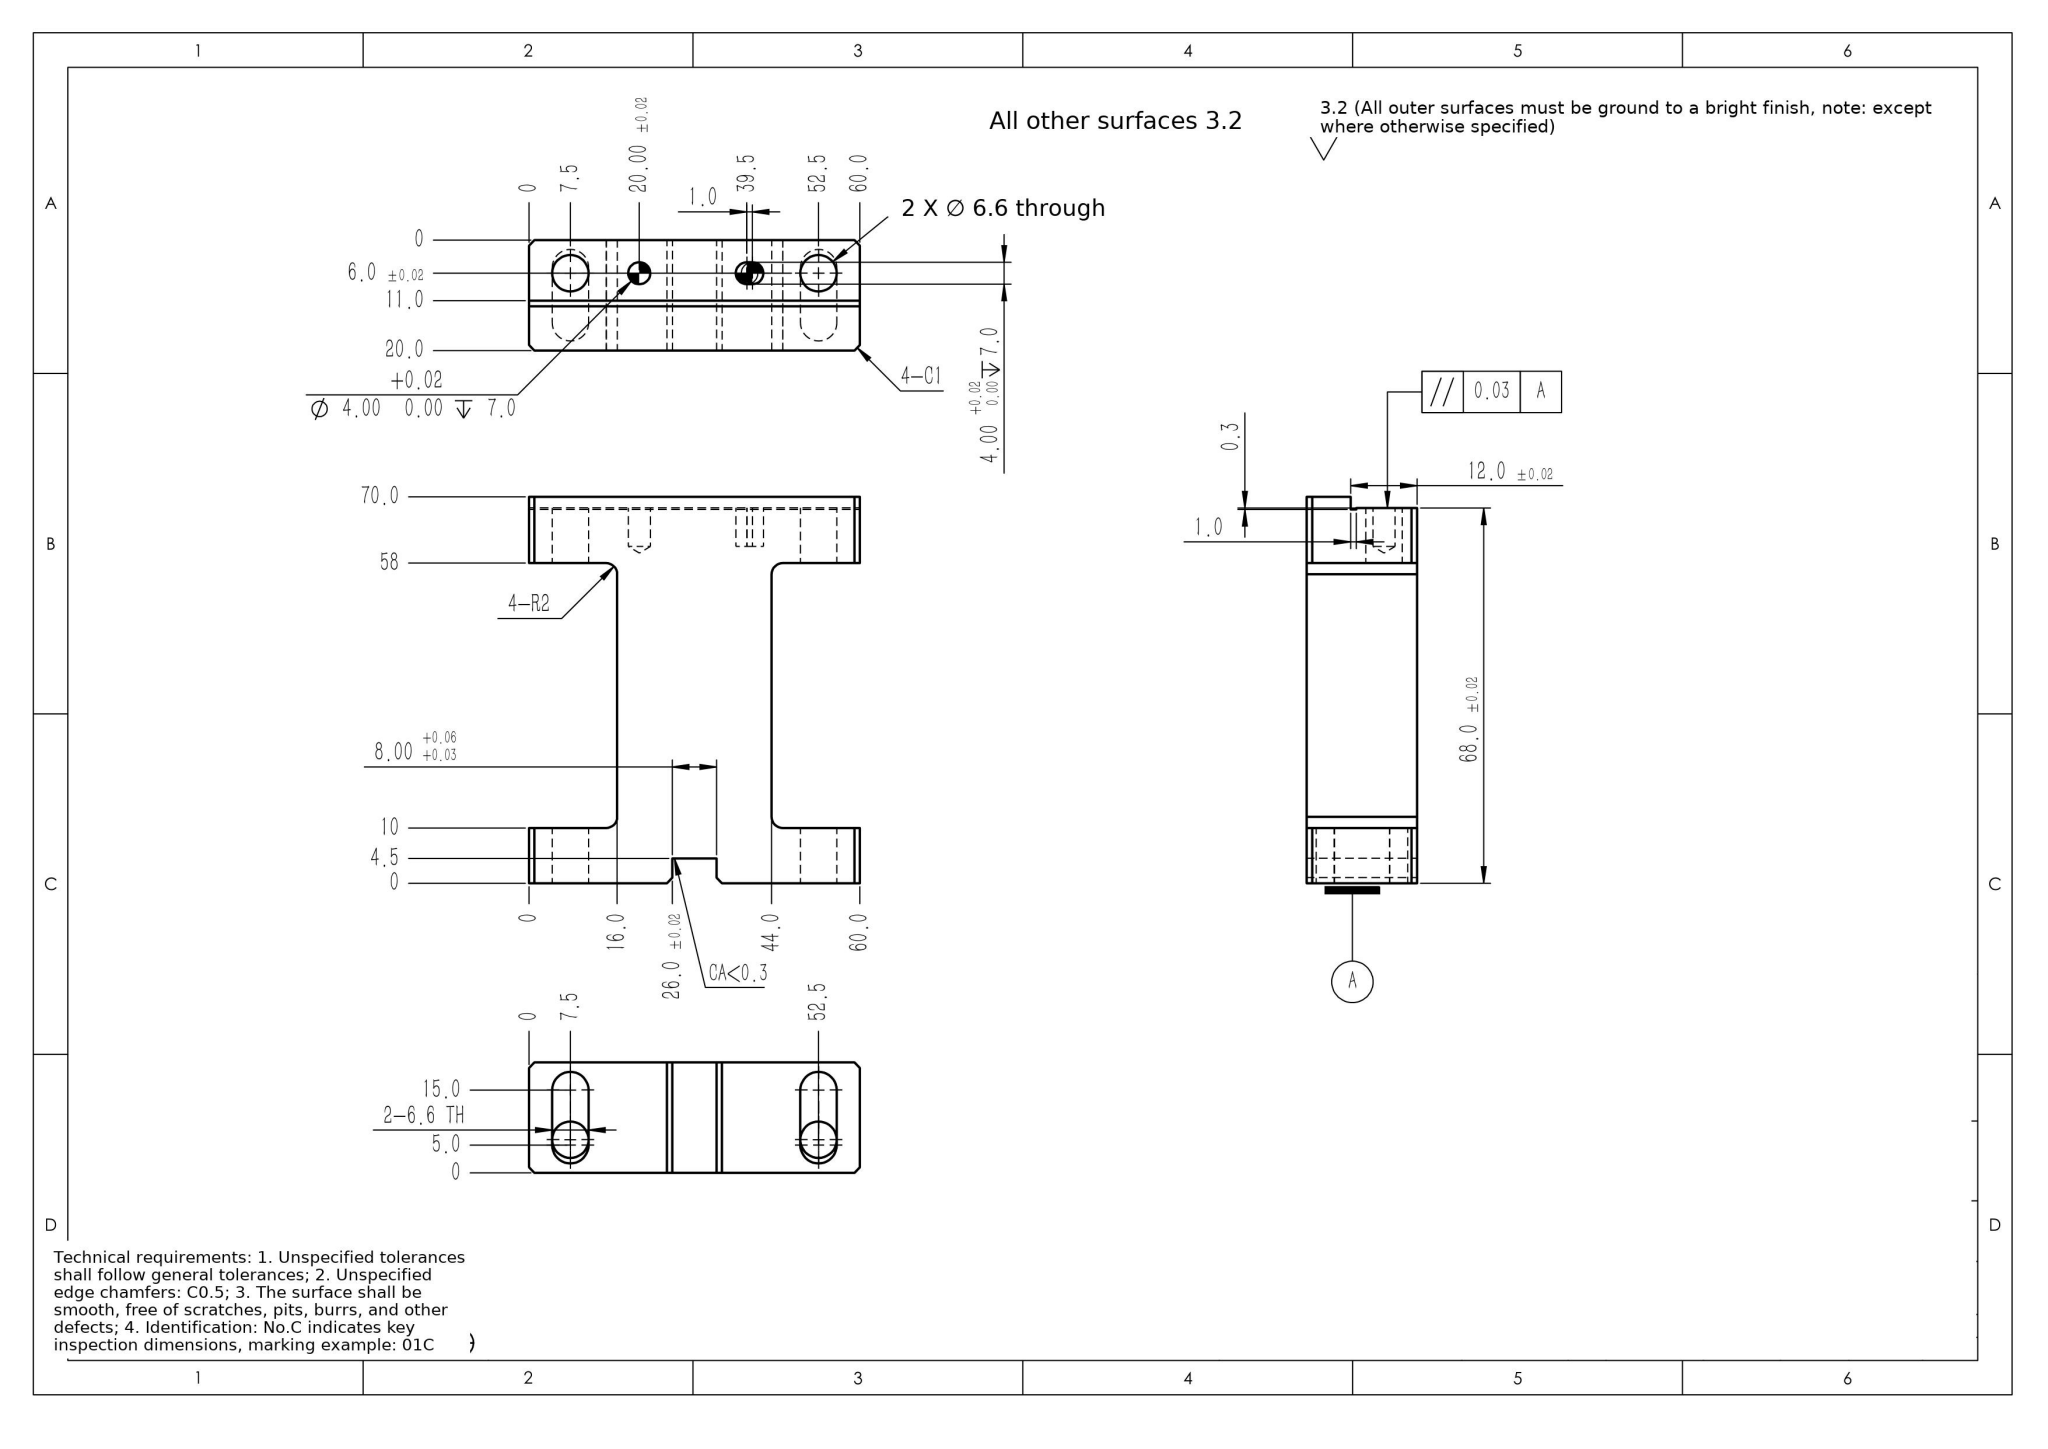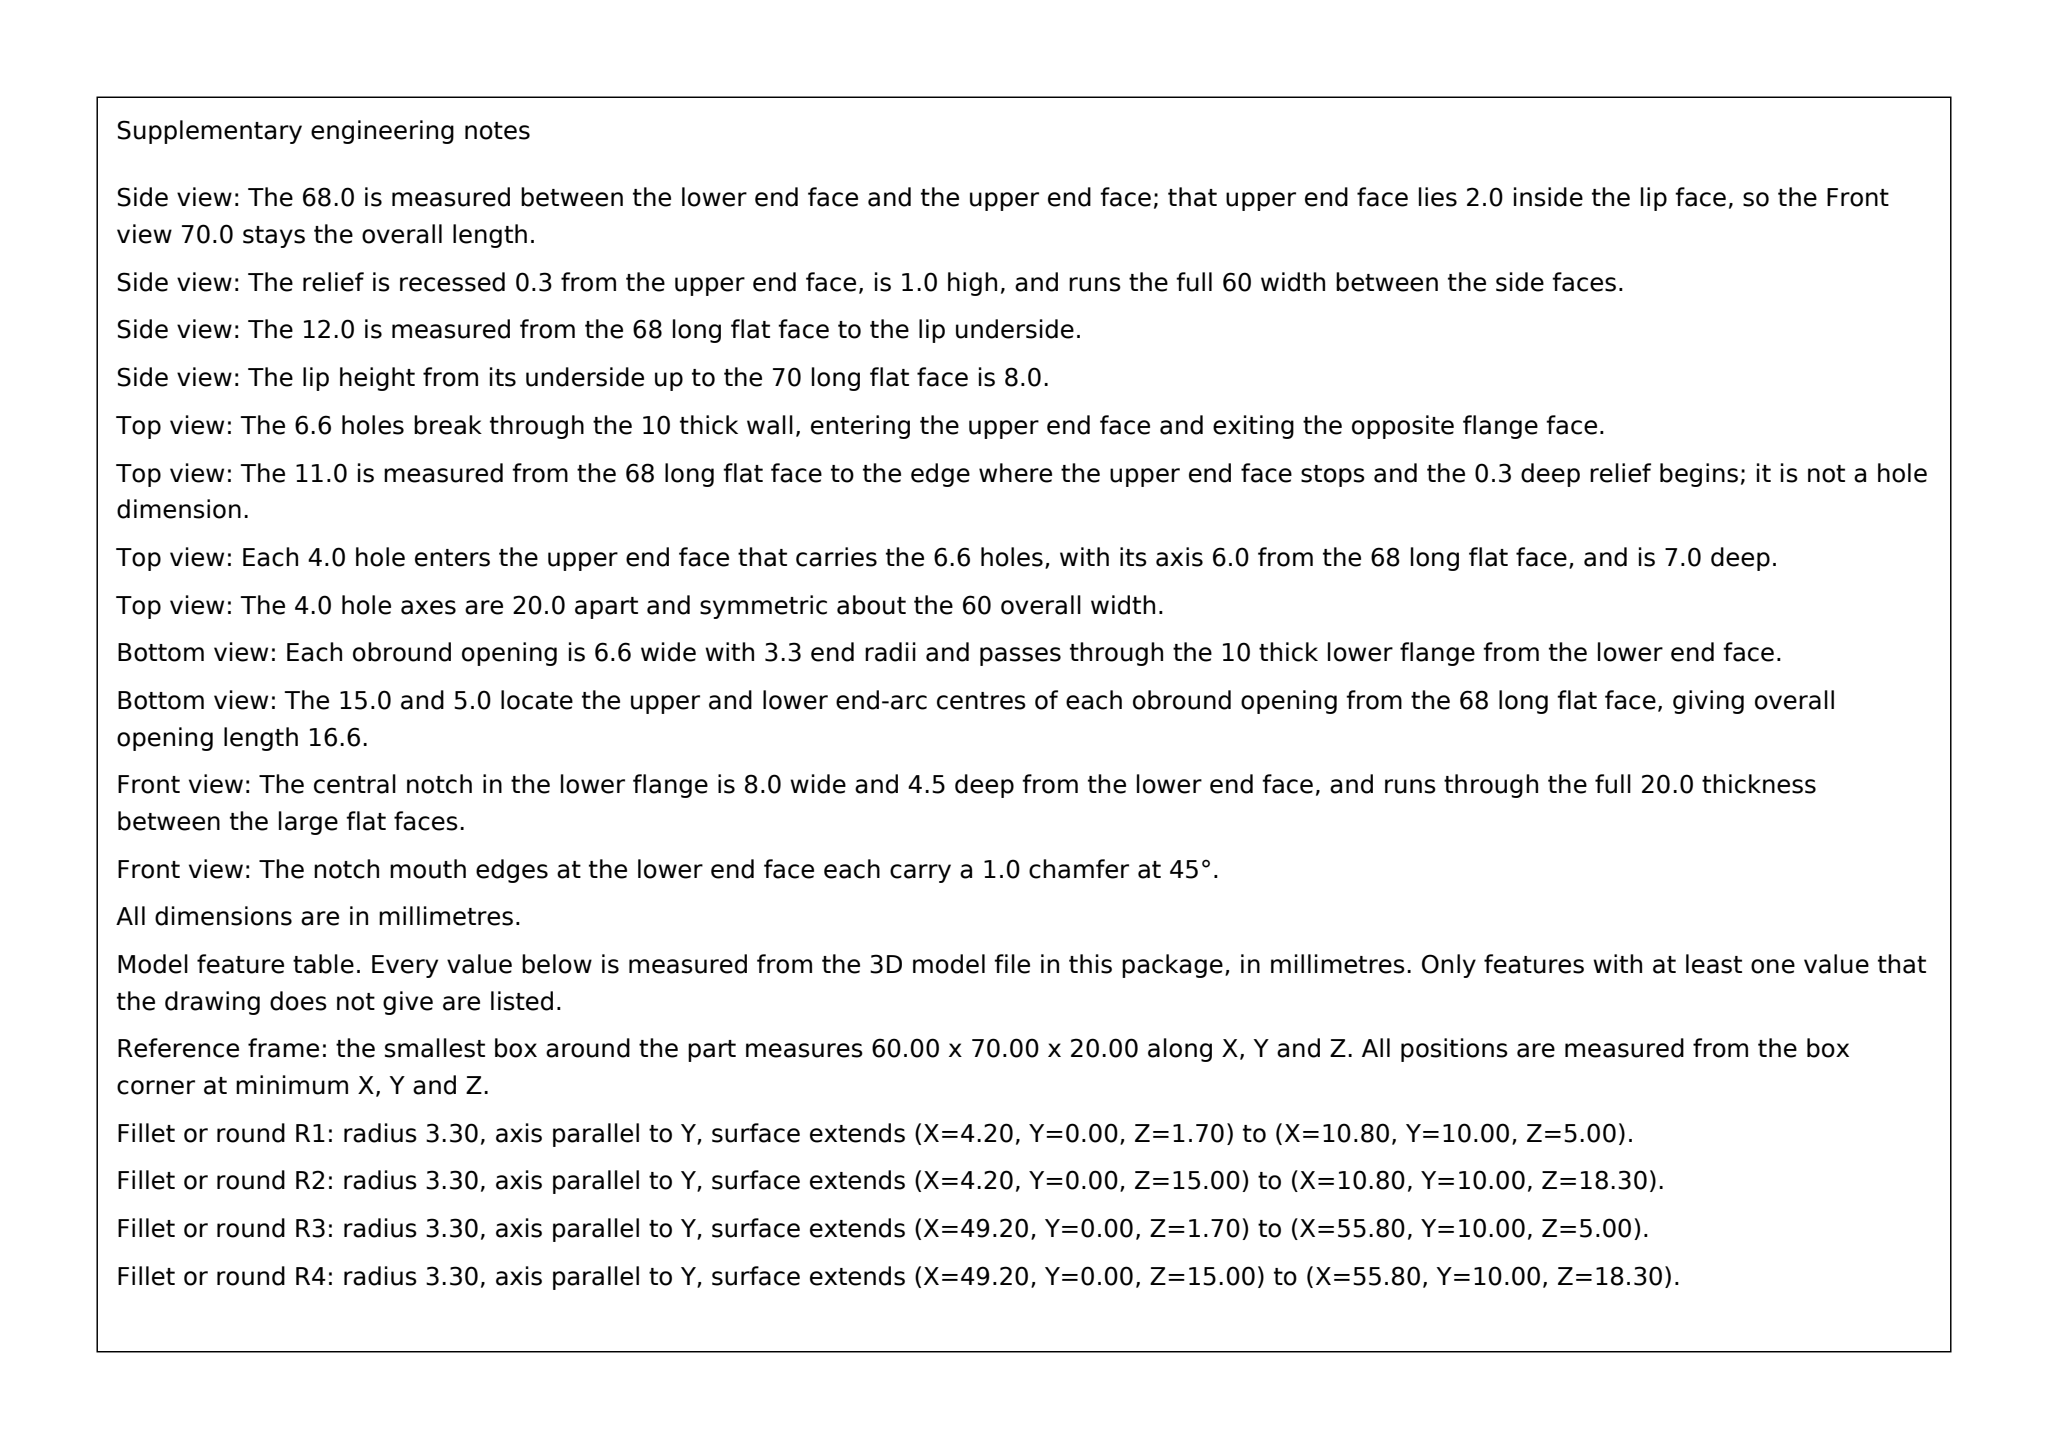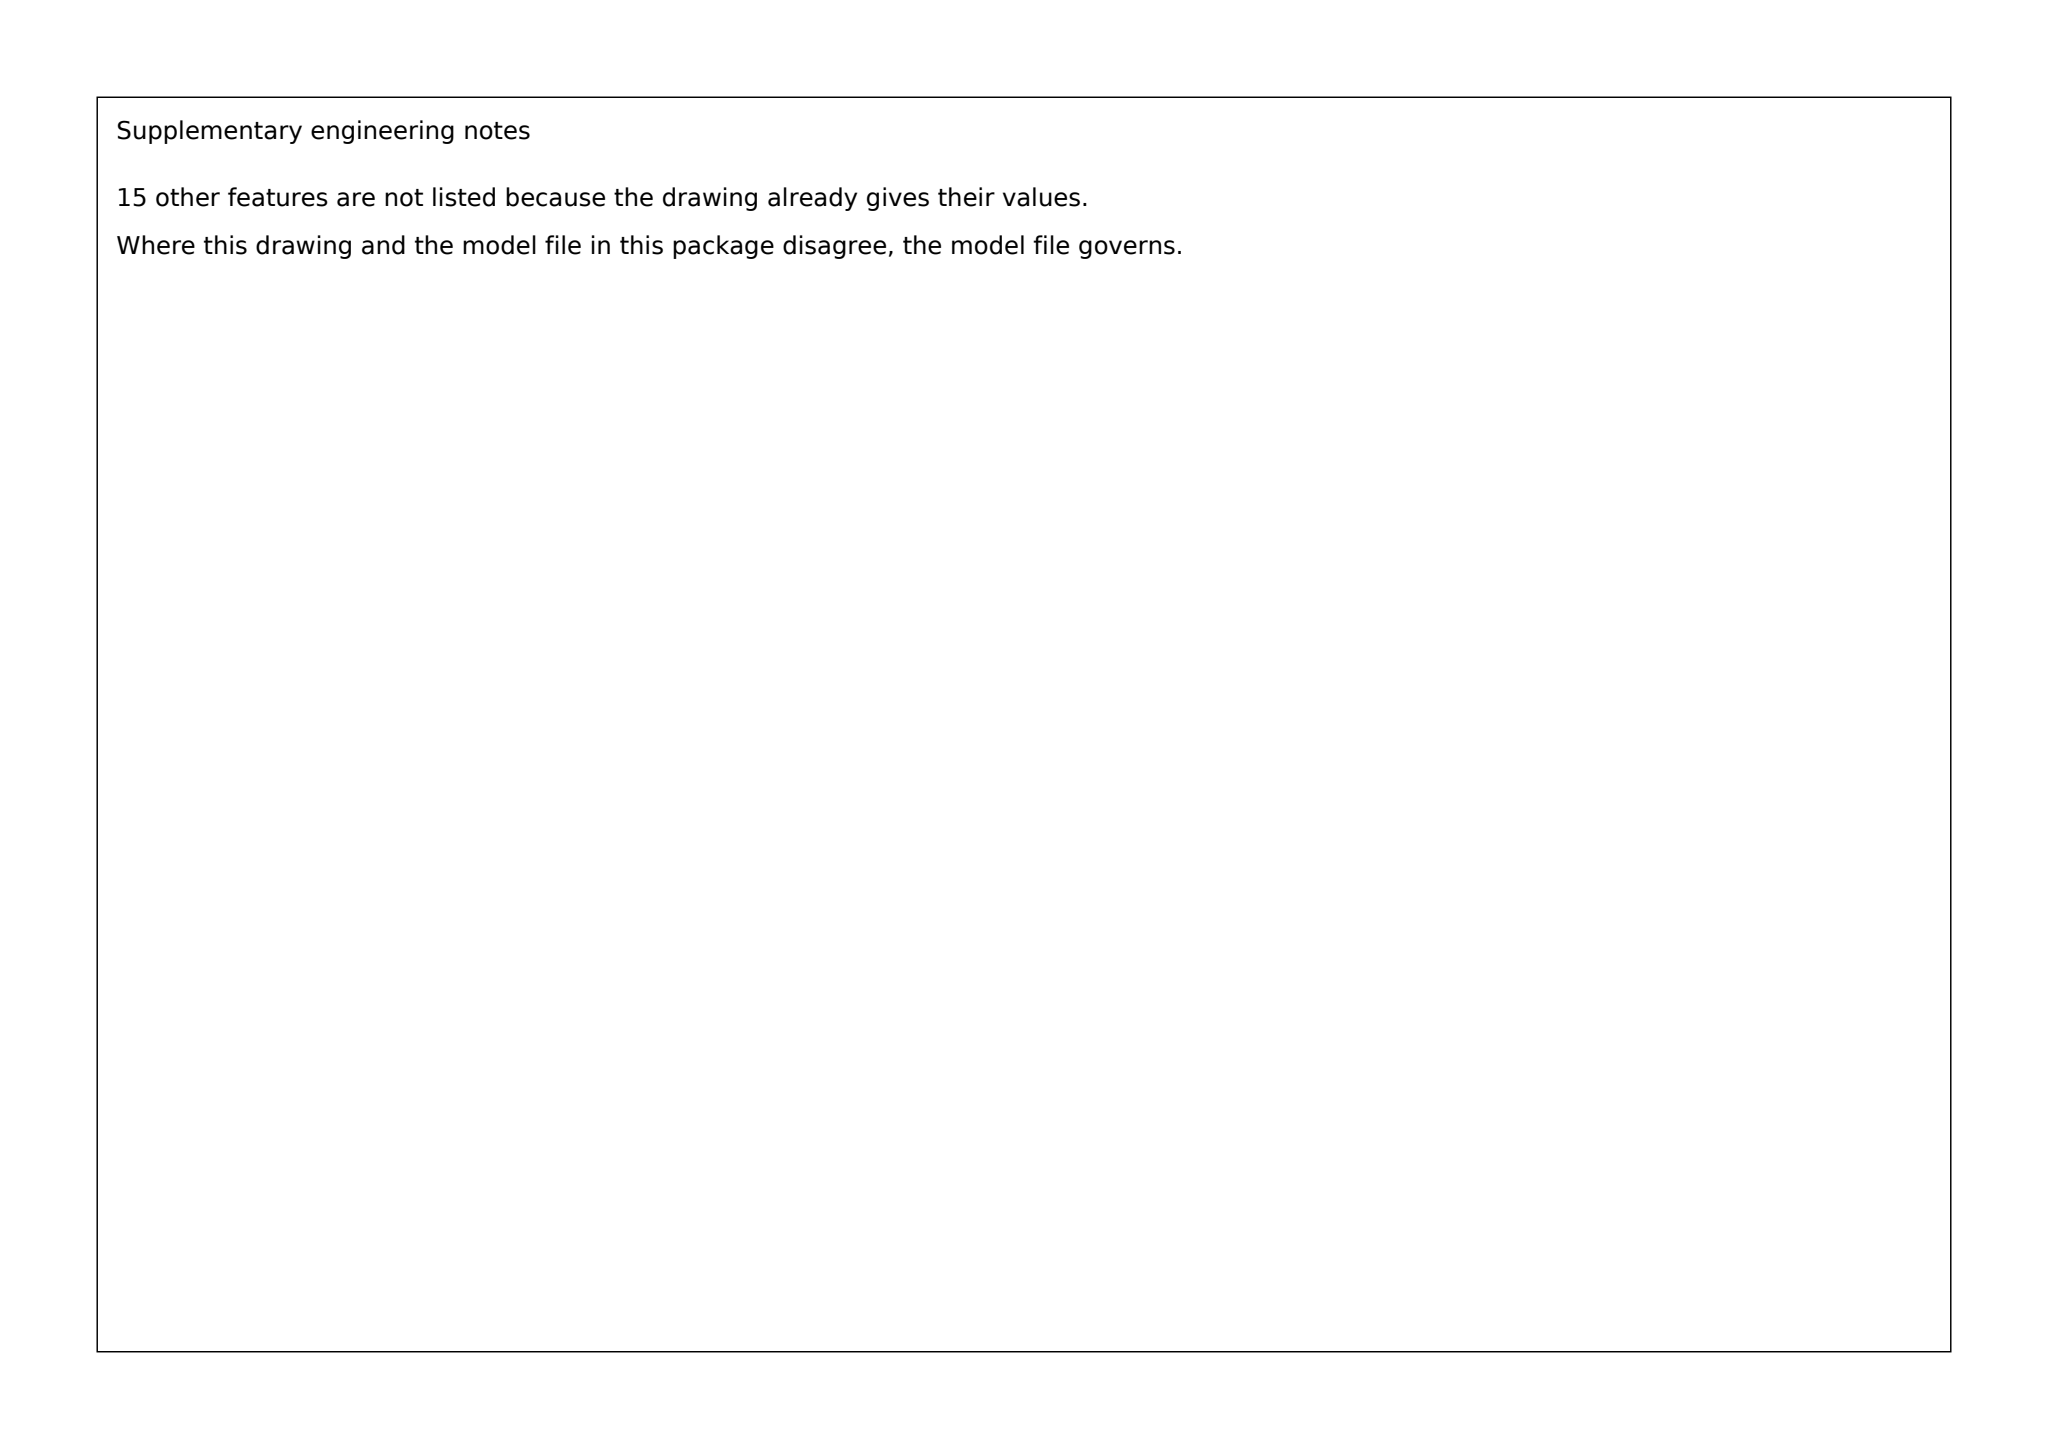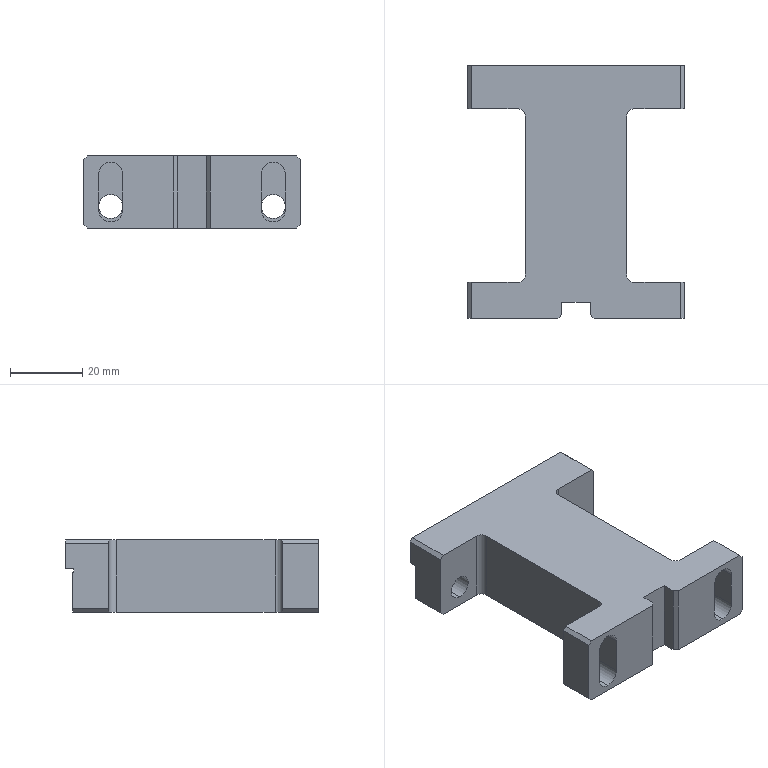Part | SolidWorks | mm | 1 solid | 59 faces | box 60 x 70 x 20 mm | volume 48211 mm3 | plane 39 | cylinder 18 | cone 2 | commonest cylinder face diameters 6.6 x10 4 x8
Drawing notes:
4X Ø4.0 THRU; X=14.0 & 46.0, Y=12.0 & 56.0 FROM 0 DATUM | from the solid: cylinders dia 4.0 axis z at (14,12),(14,56),(46,12),(46,56), length 20
4X Ø4.0 Z-AXIS HOLES THRU ALL (20.0 THK), NO C'BORE | from the solid: dia 4.0 axis z cylinders length 20.0 = full bbox z 20.0; no counterbore planes/cones on z axis
2X Ø4.00 +0.02/0 DP 7.0 AT X=20.00 & SLOT X=39.5/40.5, Z=6.0 | from the solid: dia 4.0 axis y at x=20.0 z=6.0 L7.0 (x2) and x=39.5/40.5 z=6.0 L7.0; cones 118° ref dia 4.0 x2
SLOT Ø4.00 +0.02/0 x 1.0 LG DP 7.0, CTRS X=39.5 & 40.5, Z=6.0 | from the solid: two dia 4.0 y-axis cylinders at x=39.5 and 40.5, z=6.0, length 7.0 (1.0 ctr spacing)
0.3 DEEP STEP ON TOP FACE FULL WIDTH, X=0 TO 60.0 | from the solid: y planes 68.0 and 67.7 (0.3 apart); no intermediate x planes besides slot walls, bbox x=60.0
build123d program:
from build123d import *

# Parameters (mm, degrees)
SKETCH2_W                      = 60
SKETCH2_H                      = 68
BOSS_EXTRUDE1_DEPTH            = 20
SKETCH3_W                      = 16
SKETCH3_H                      = 48
CUT_EXTRUDE1_DEPTH             = 20
F_6_6_6_6_DIAMETER_HOLE2_D     = 6.6
F_6_6_6_6_DIAMETER_HOLE2_DEPTH = 10
SIZE_MM_DOWEL_PIN_HOLE_1_D     = 4
SIZE_MM_DOWEL_PIN_HOLE_1_DEPTH = 7
SIZE_MM_DOWEL_PIN_HOLE_1_TIP   = 1.202
CUT_EXTRUDE2_DEPTH             = 7
SKETCH18_W                     = 8
SKETCH18_H                     = 4.5
CUT_EXTRUDE5_DEPTH             = 50.558
SKETCH19_W                     = 60
SKETCH19_H                     = 8
BOSS_EXTRUDE4_DEPTH            = 2
SKETCH20_W                     = 1
SKETCH20_H                     = 0.3
CUT_EXTRUDE6_DEPTH             = 73.774
CUT_EXTRUDE7_REACH             = 80.74
CHAMFER1_SIZE                  = 1
FILLET1_R                      = 2


with BuildPart() as part:
    # Sketch2 → Boss-Extrude1 (new body)
    with BuildSketch(Plane.XY):
        Rectangle(SKETCH2_W, SKETCH2_H)
    extrude(amount=BOSS_EXTRUDE1_DEPTH)

    # Sketch3 → Cut-Extrude1 (cut)
    with BuildSketch(Plane.XY.offset(20)):
        with Locations((-22, 0)):
            Rectangle(SKETCH3_W, SKETCH3_H)
        with Locations((22, 0)):
            Rectangle(SKETCH3_W, SKETCH3_H)
    extrude(amount=-CUT_EXTRUDE1_DEPTH, mode=Mode.SUBTRACT)

    # 6.6 _6.6_ Diameter Hole2
    with Locations(Plane(origin=(0, 34, 0), x_dir=(1, 0, 0), z_dir=(0, 1, 0))):
        with Locations((-22.5, -6), (22.5, -6)):
            Hole(F_6_6_6_6_DIAMETER_HOLE2_D / 2, depth=F_6_6_6_6_DIAMETER_HOLE2_DEPTH)

    # Size mm Dowel Pin Hole 1
    with Locations(Plane(origin=(0, 34, 0), x_dir=(1, 0, 0), z_dir=(0, 1, 0))):
        with Locations((-10, -6)):
            Hole(SIZE_MM_DOWEL_PIN_HOLE_1_D / 2, depth=SIZE_MM_DOWEL_PIN_HOLE_1_DEPTH)
            with Locations((0, 0, -(SIZE_MM_DOWEL_PIN_HOLE_1_DEPTH + SIZE_MM_DOWEL_PIN_HOLE_1_TIP / 2))):  # 118° drill point
                Cone(0, SIZE_MM_DOWEL_PIN_HOLE_1_D / 2, SIZE_MM_DOWEL_PIN_HOLE_1_TIP, mode=Mode.SUBTRACT)

    # Sketch8 → Cut-Extrude2 (cut)
    with BuildSketch(Plane(origin=(0, 34, 0), x_dir=(1, 0, 0), z_dir=(0, 1, 0))):
        with BuildLine():
            Line((9.5, -4), (10.5, -4))
            ThreePointArc((10.5, -4), (12.5, -6), (10.5, -8))
            Line((10.5, -8), (9.5, -8))
            ThreePointArc((9.5, -8), (7.5, -6), (9.5, -4))
        make_face()
    extrude(amount=-CUT_EXTRUDE2_DEPTH, mode=Mode.SUBTRACT)

    # Sketch18 → Cut-Extrude5 (cut, through all)
    with BuildSketch(Plane.XY.offset(20)):
        with Locations((0, -31.75)):
            Rectangle(SKETCH18_W, SKETCH18_H)
    extrude(amount=-CUT_EXTRUDE5_DEPTH, mode=Mode.SUBTRACT)

    # Sketch19 → Boss-Extrude4 (add)
    with BuildSketch(Plane(origin=(0, 34, 0), x_dir=(1, 0, 0), z_dir=(0, 1, 0))):
        with Locations((0, -16)):
            Rectangle(SKETCH19_W, SKETCH19_H)
    extrude(amount=BOSS_EXTRUDE4_DEPTH)

    # Sketch20 → Cut-Extrude6 (cut, through all)
    with BuildSketch(Plane(origin=(30, 0, 0), x_dir=(0, 0, -1), z_dir=(1, 0, 0))):
        with Locations((-11.5, 33.85)):
            Rectangle(SKETCH20_W, SKETCH20_H)
    extrude(amount=-CUT_EXTRUDE6_DEPTH, mode=Mode.SUBTRACT)

    # Sketch22 → Cut-Extrude7 (cut, up to next)
    with BuildSketch(Plane.XZ.offset(34), mode=Mode.PRIVATE) as cut_extrude7_sk1:
        with BuildLine():
            Line((-19.2, 15), (-19.2, 5))
            ThreePointArc((-19.2, 5), (-22.5, 1.7), (-25.8, 5))
            Line((-25.8, 5), (-25.8, 15))
            ThreePointArc((-25.8, 15), (-22.5, 18.3), (-19.2, 15))
        make_face()
    cut_extrude7_tool1 = extrude(cut_extrude7_sk1.sketch, amount=-CUT_EXTRUDE7_REACH, mode=Mode.PRIVATE) & part.part
    # Sketch22 → Cut-Extrude7 (cut, up to next)
    with BuildSketch(Plane.XZ.offset(34), mode=Mode.PRIVATE) as cut_extrude7_sk2:
        with BuildLine():
            Line((25.8, 15), (25.8, 5))
            ThreePointArc((25.8, 5), (22.5, 1.7), (19.2, 5))
            Line((19.2, 5), (19.2, 15))
            ThreePointArc((19.2, 15), (22.5, 18.3), (25.8, 15))
        make_face()
    cut_extrude7_tool2 = extrude(cut_extrude7_sk2.sketch, amount=-CUT_EXTRUDE7_REACH, mode=Mode.PRIVATE) & part.part
    add(cut_extrude7_tool1.solids().sort_by_distance((-22.5, -34, 10))[0], mode=Mode.SUBTRACT)
    add(cut_extrude7_tool2.solids().sort_by_distance((22.5, -34, 10))[0], mode=Mode.SUBTRACT)

    # Chamfer1
    chamfer1_edges = [part.edges().sort_by_distance(p)[0] for p in [
        (30, 30, 20),
        (-30, -29, 0),
        (-30, -29, 20),
        (30, -29, 0),
        (30, -29, 20),
        (-30, 30, 20),
        (30, 29, 0),
        (-30, 29, 0),
        (-4, -34, 10),
        (4, -34, 10),
    ]]
    chamfer(chamfer1_edges, length=CHAMFER1_SIZE)

    # Fillet1
    fillet1_edges = [part.edges().sort_by_distance(p)[0] for p in [
        (-14, 24, 10),
        (-14, -24, 10),
        (14, -24, 10),
        (14, 24, 10),
    ]]
    fillet(fillet1_edges, radius=FILLET1_R)


solid = part.part